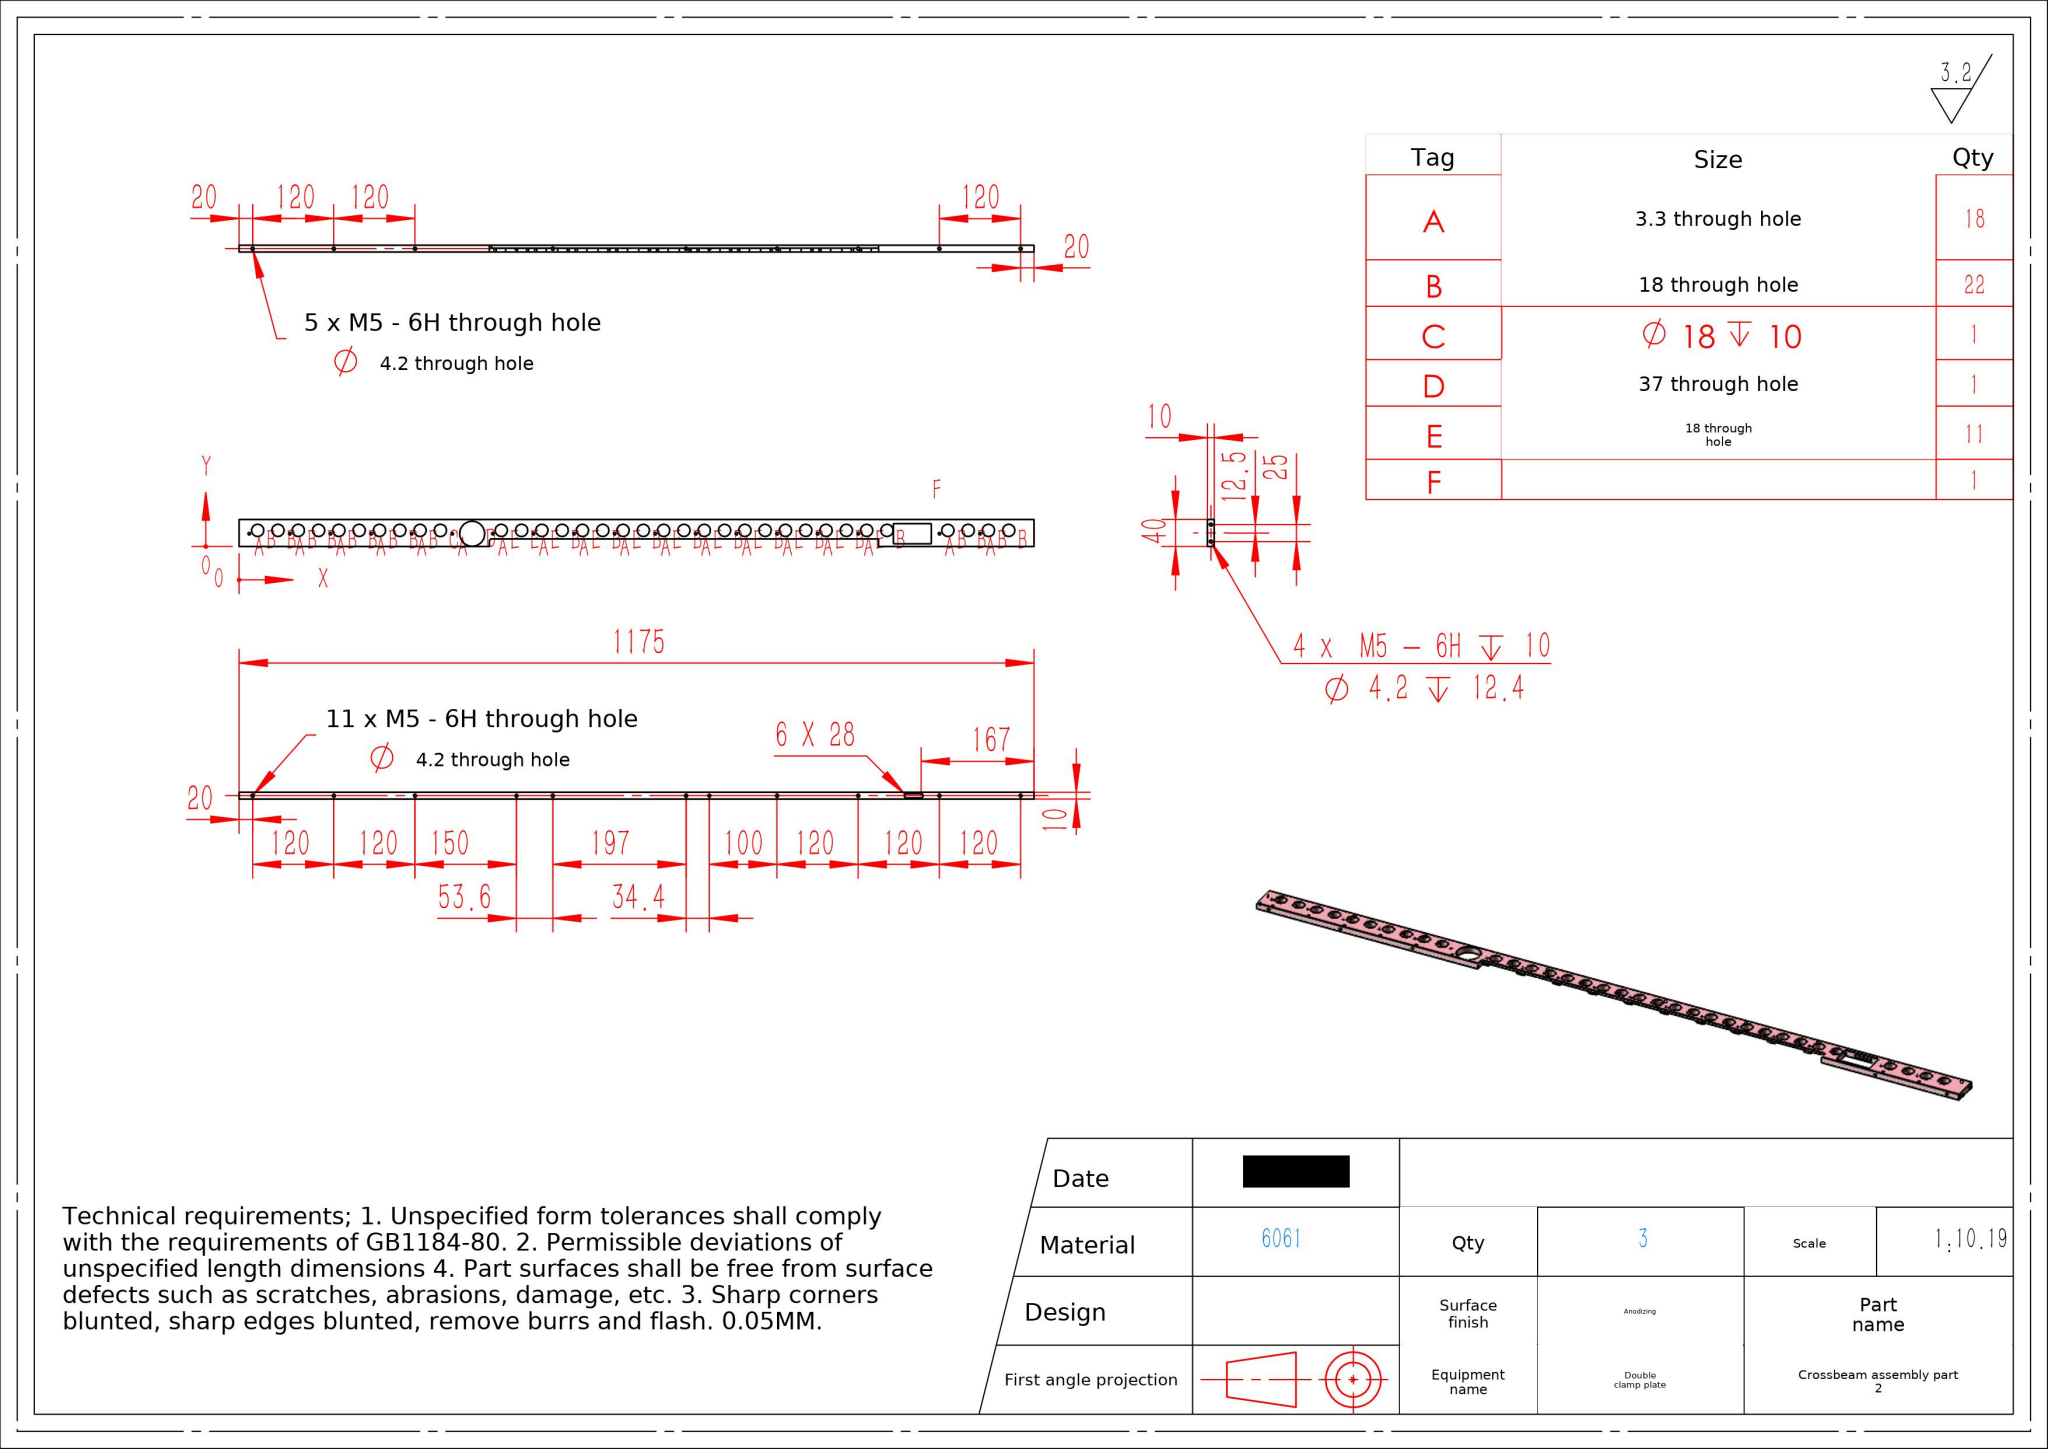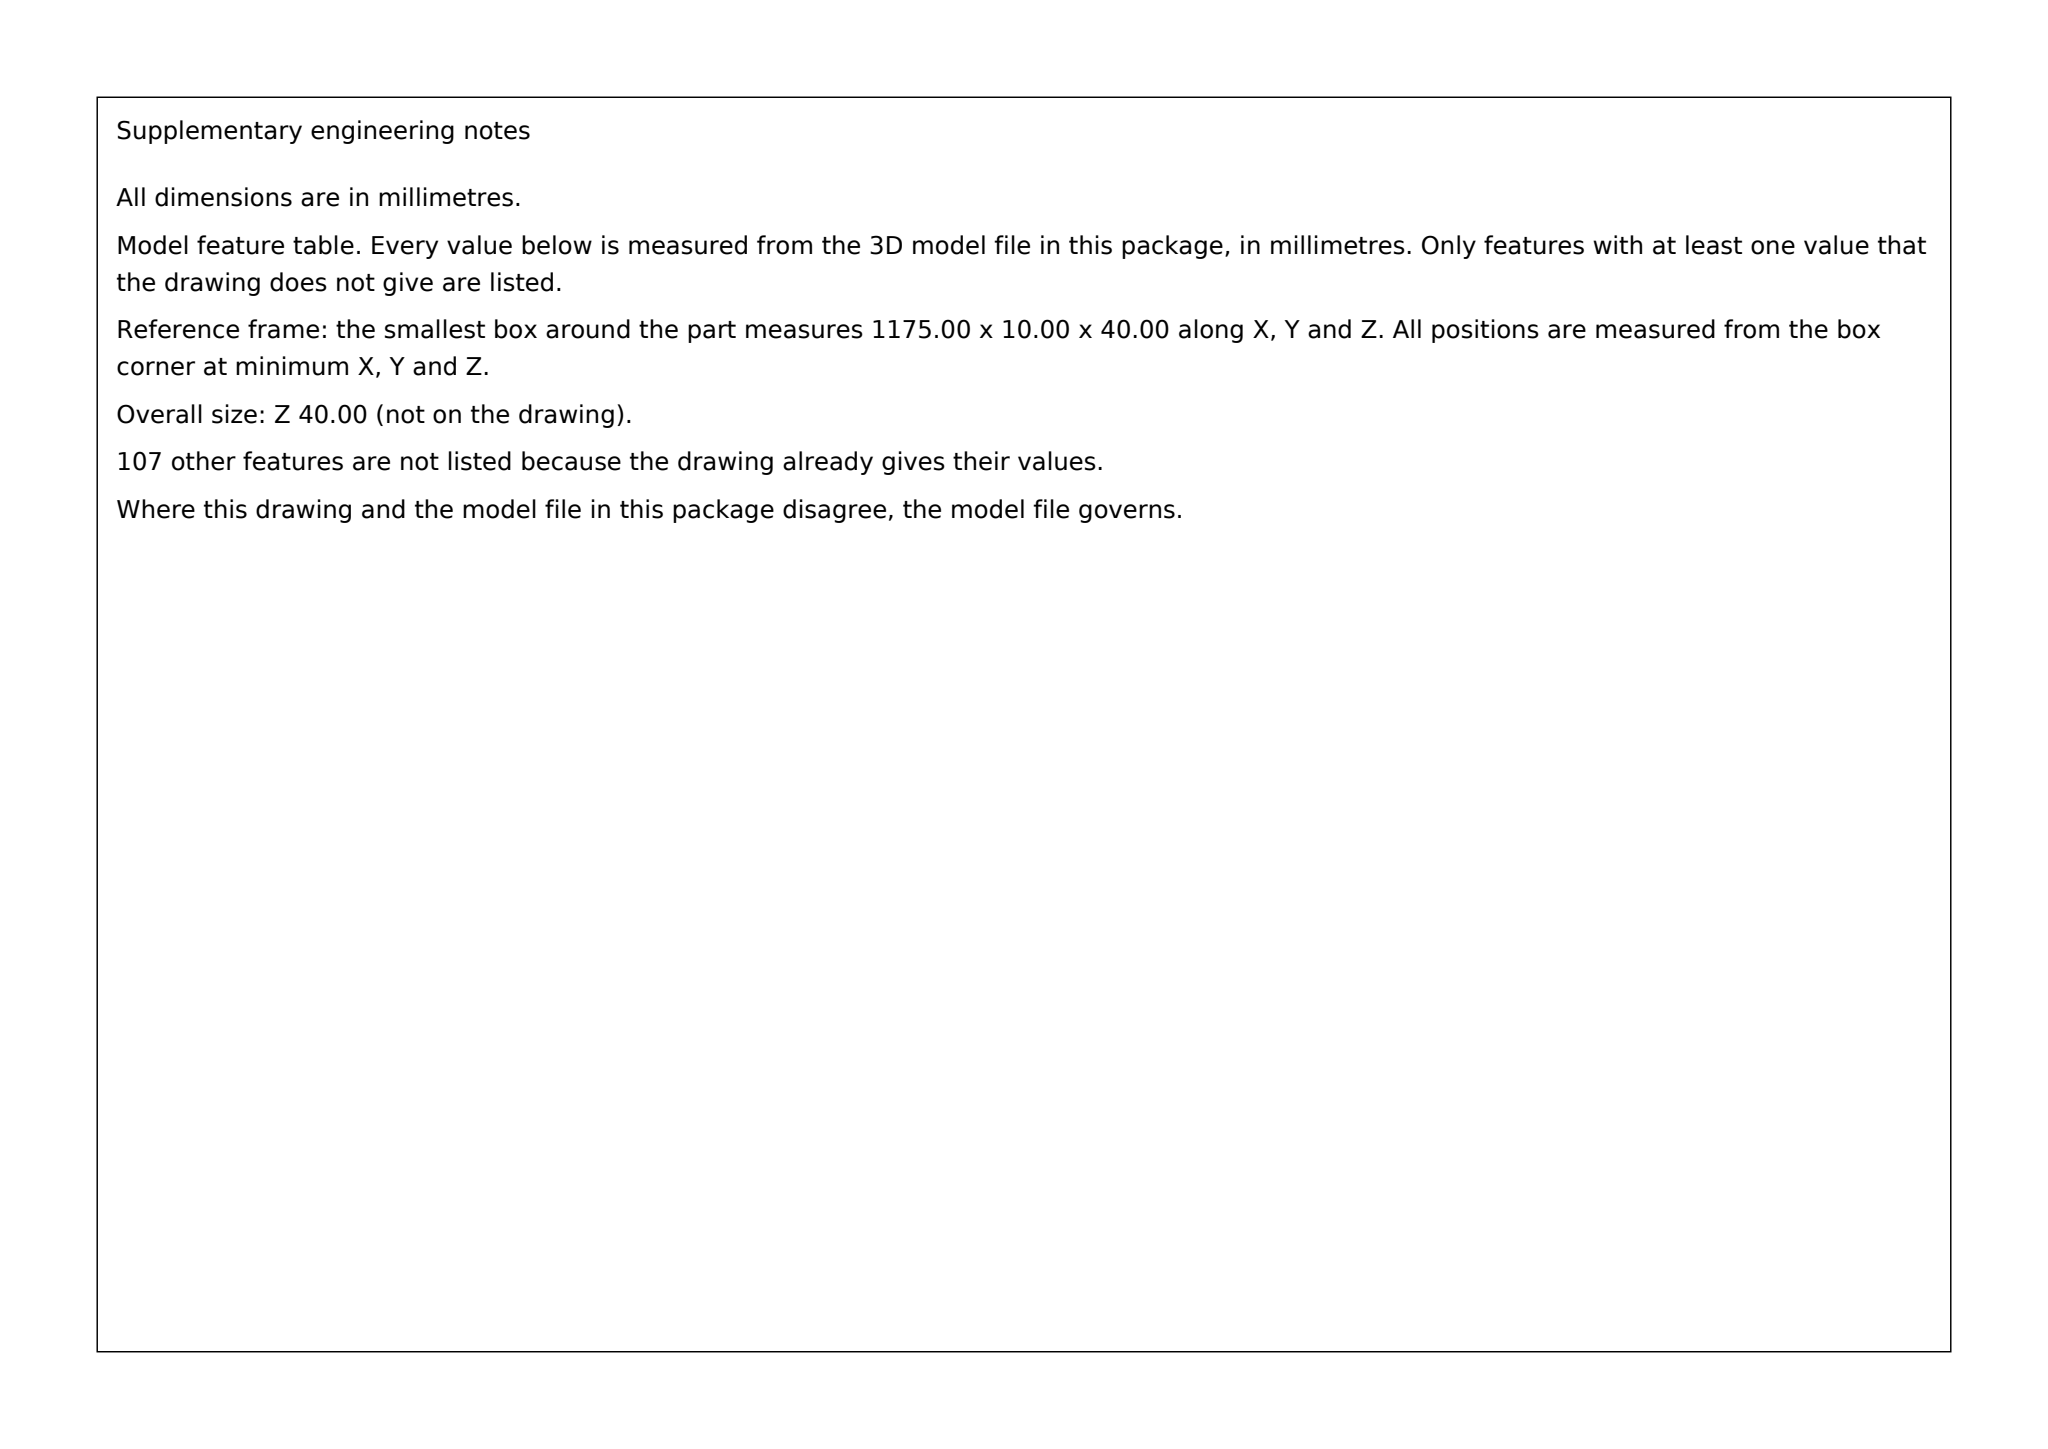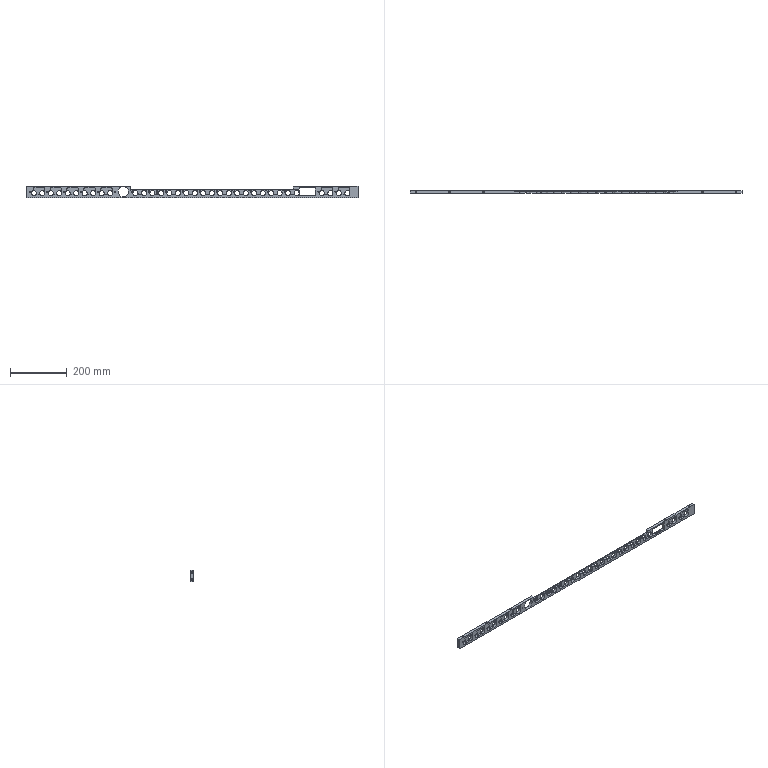Part | SolidWorks | mm | material 6061 | 1 solid | 282 faces | box 1175 x 10 x 40 mm | volume 229708 mm3 | cylinder 184 | plane 88 | cone 10 | commonest cylinder face diameters 18 x68 3.3 x42 6 x37 4.2 x30 2 x4 37 x2 10 x1